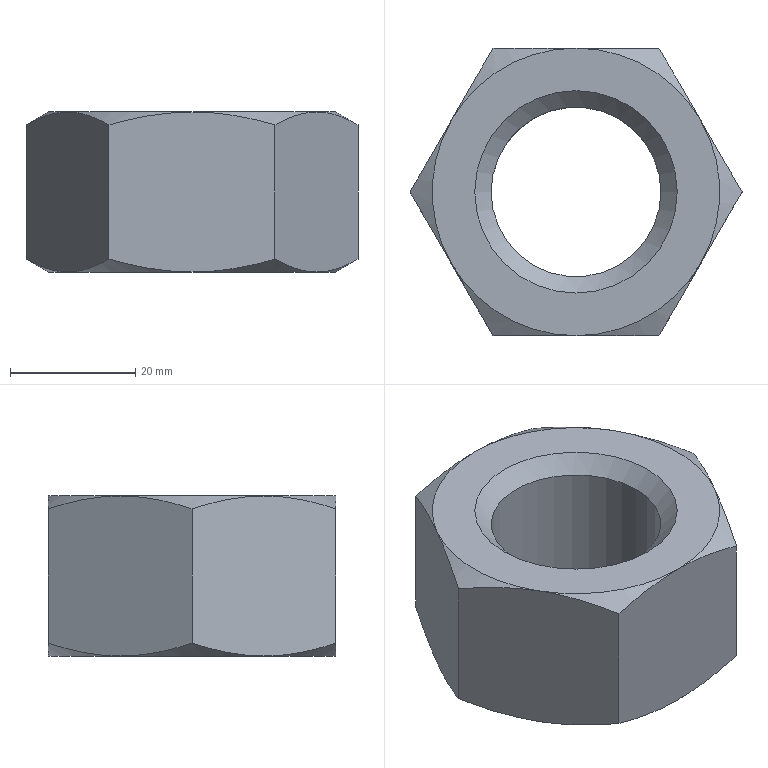Component | NX | GB-T6170_F-2000_M30X3_5_2 | 1 solid | 23 faces | volume 31247 mm3 | cone 14 | plane 8 | cylinder 1 | commonest cylinder face diameters 27.158 x1